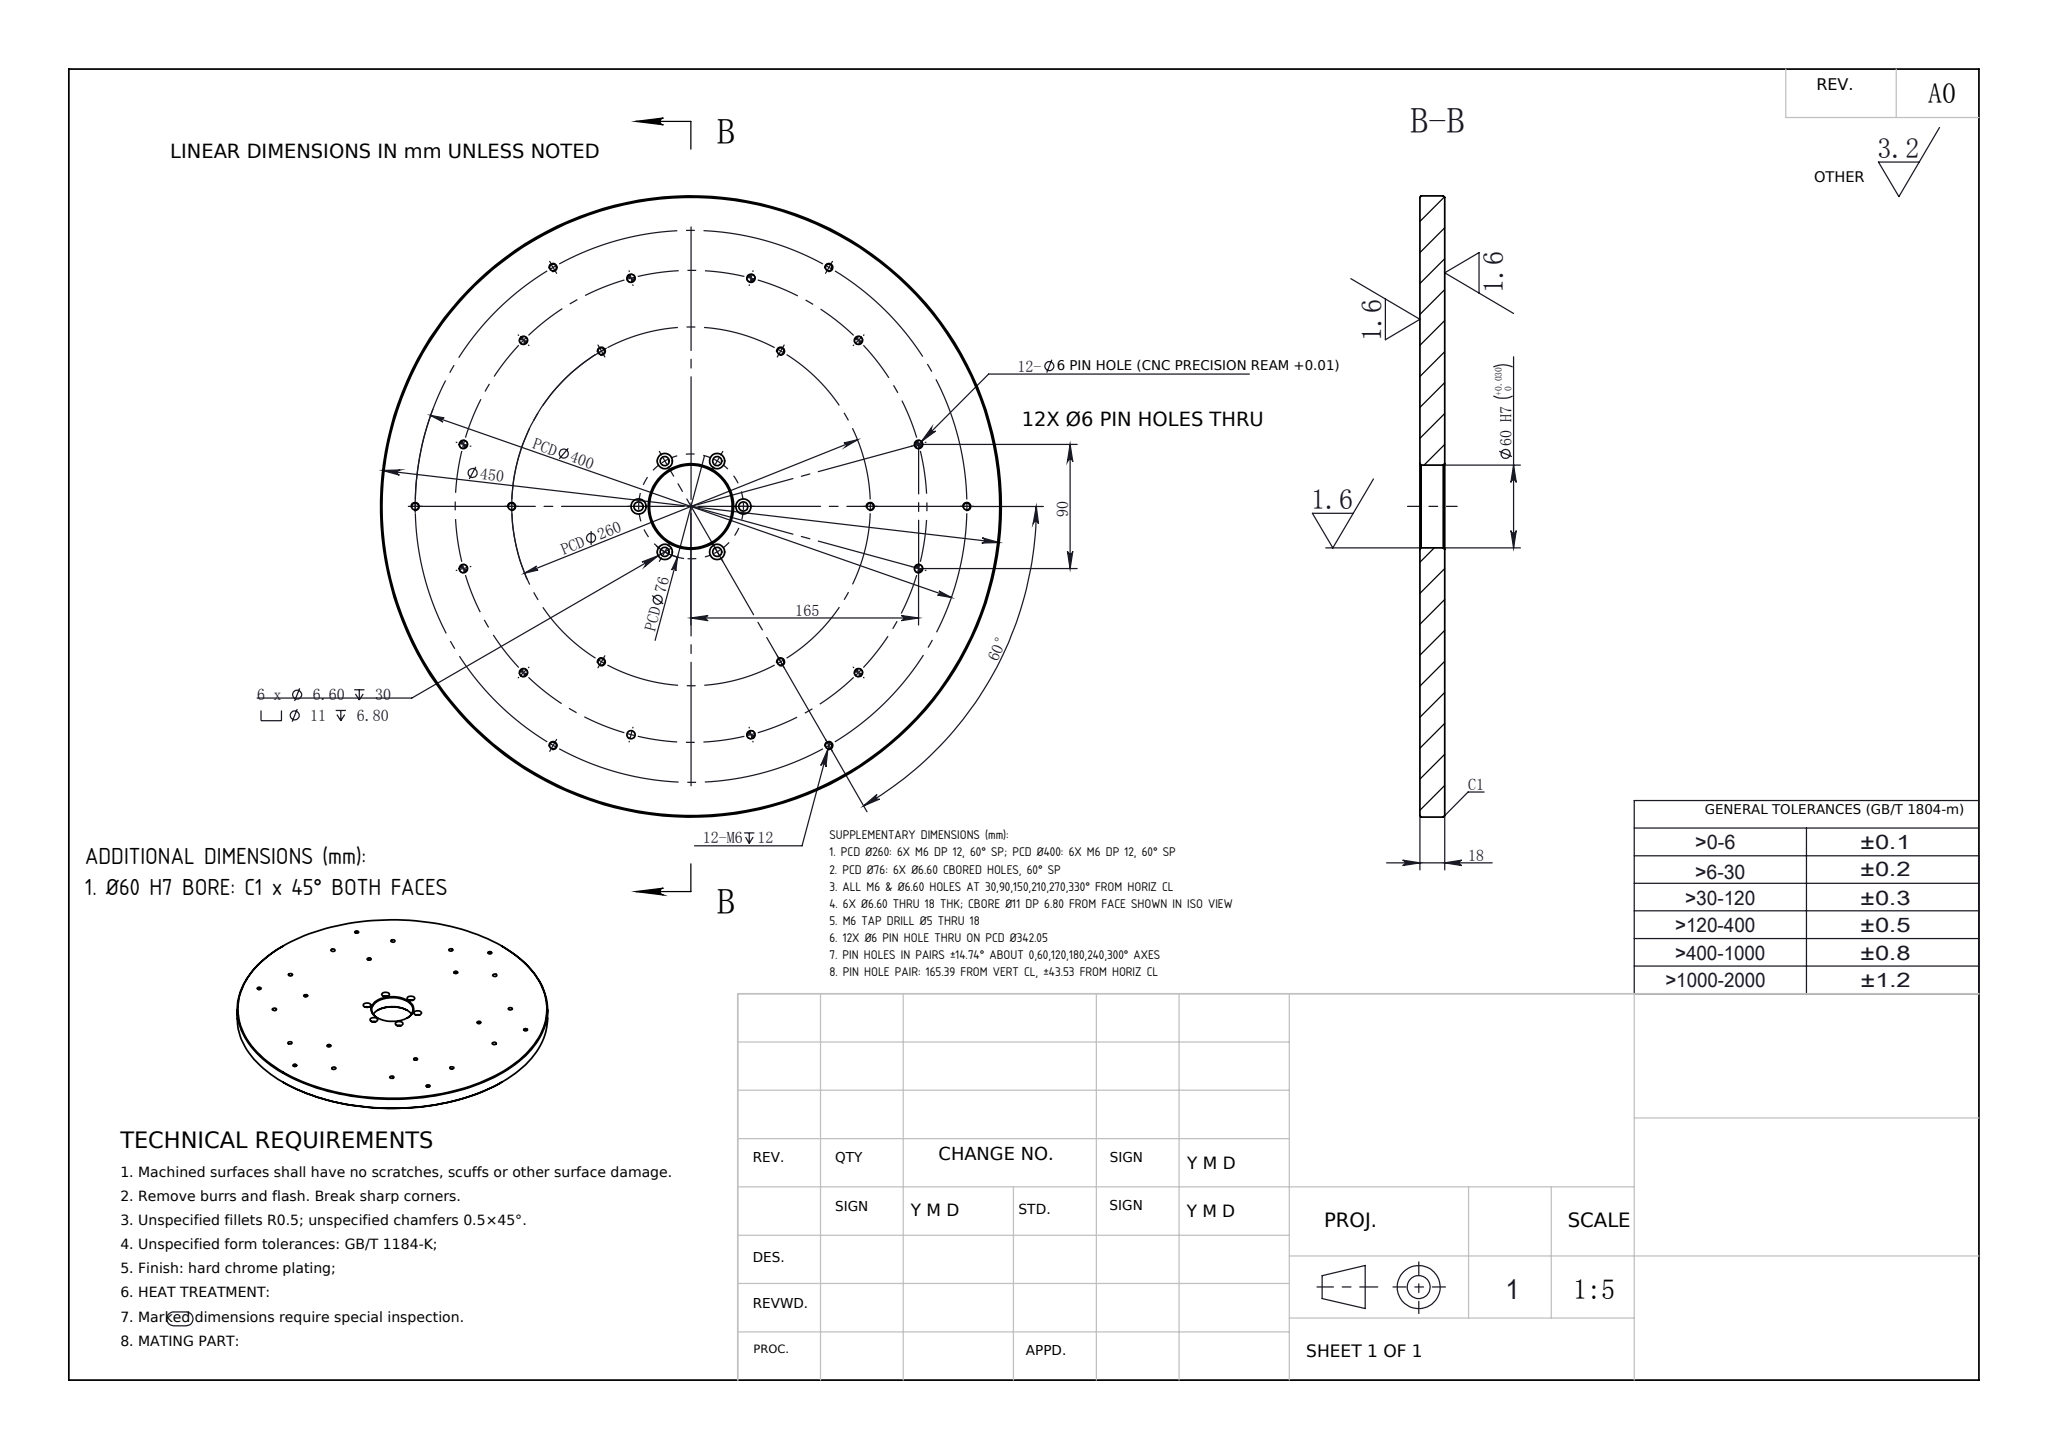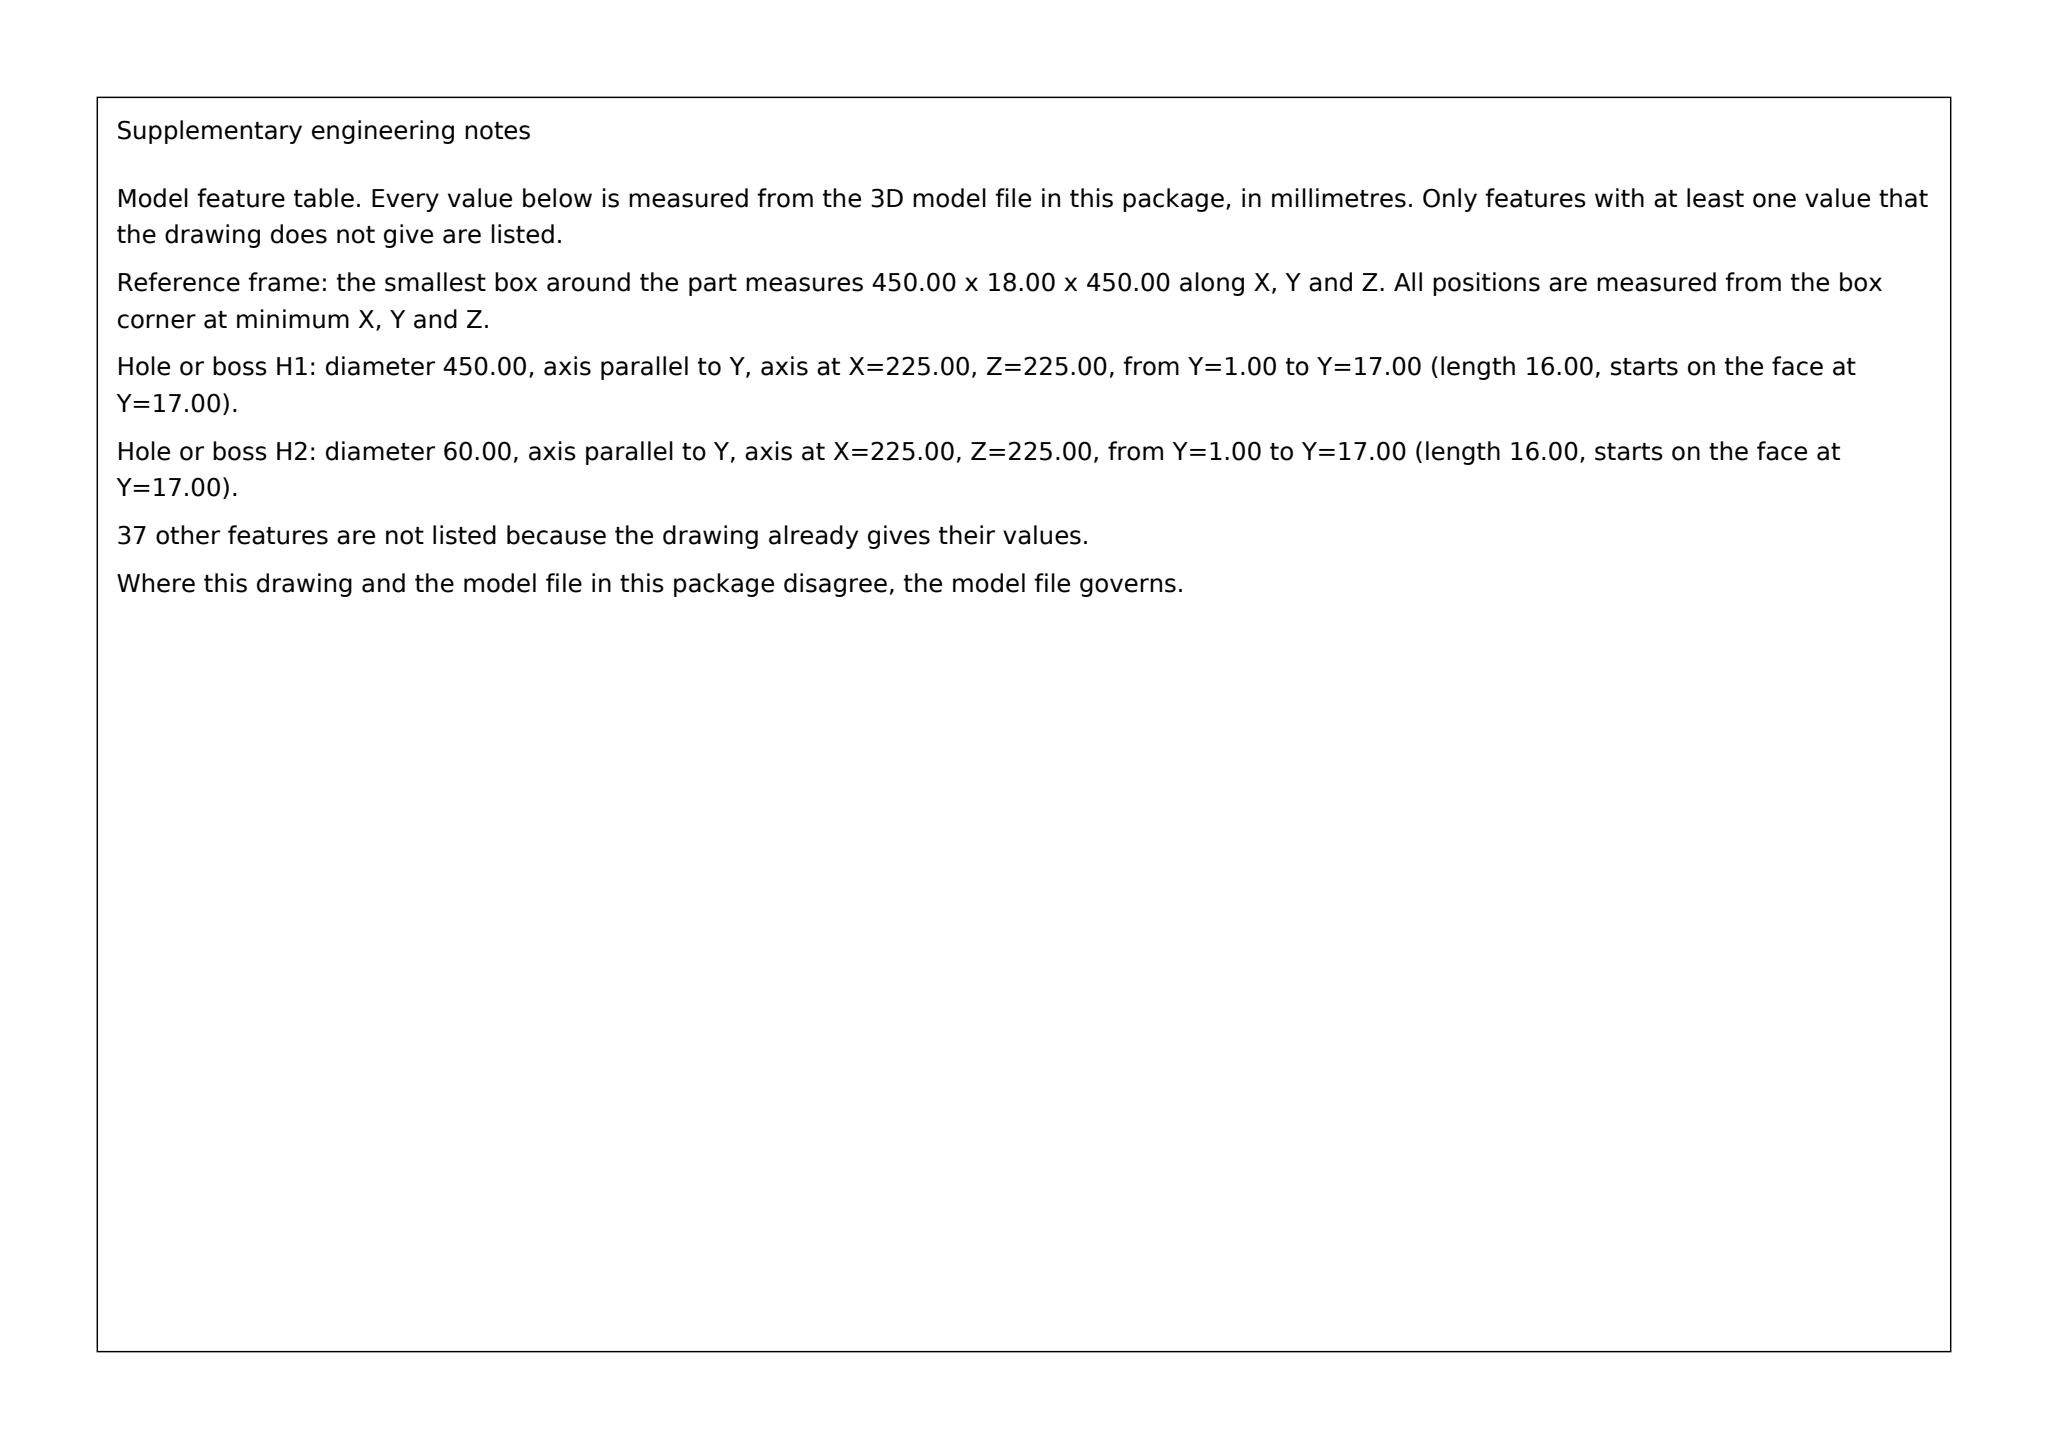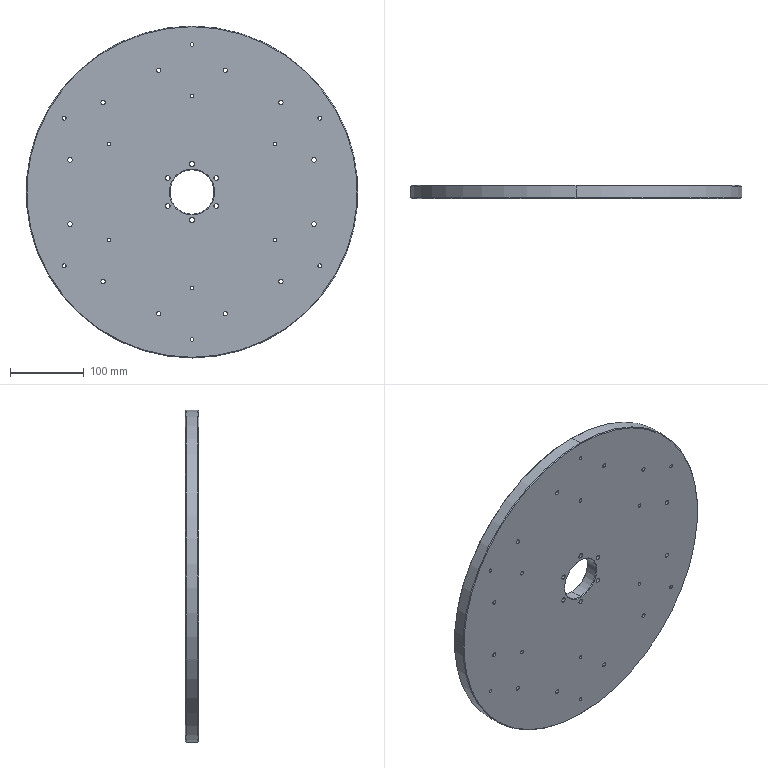Part | SolidWorks | mm | 1 solid | 92 faces | box 450 x 18 x 450 mm | volume 2793755 mm3 | cylinder 76 | cone 8 | plane 8 | commonest cylinder face diameters 5 x24 6 x24 11 x12 6.6 x12 60 x2 450 x2
build123d program:
from build123d import *

# Parameters (mm, degrees)
SKETCH1_R                  = 225
EXTRUDE1_DEPTH             = 18
SKETCH2_R                  = 3
CUT_EXTRUDE1_DEPTH         = 319.707
CIRPATTERN1_COUNT          = 6
SKETCH3_R                  = 30
EXTRUDE2_DEPTH             = 319.707
M6_TAPPED_HOLE1_AT_2_COUNT = 2
M6_TAPPED_HOLE1_AT_2_PITCH = 70
CIRPATTERN2_COUNT          = 6
CHAMFER1_SIZE              = 1
CIRPATTERN3_COUNT          = 6


with BuildPart() as part:
    # Sketch1 → Extrude1 (new body)
    with BuildSketch(Plane(origin=(0, 0, 0), x_dir=(1, 0, 0), z_dir=(0, 1, 0))):
        with Locations(Location((0, 0, 0), (0, 0, 270))):
            Circle(SKETCH1_R)
    extrude(amount=EXTRUDE1_DEPTH)

    # Sketch2 → Cut-Extrude1 (cut, through all)
    with BuildSketch(Plane(origin=(0, 18, 0), x_dir=(1, 0, 0), z_dir=(0, 1, 0))):
        with Locations(Location((-45, -165, 0), (0, 0, 270))):
            Circle(SKETCH2_R)
        with Locations(Location((45, -165, 0), (0, 0, 270))):
            Circle(SKETCH2_R)
    cut_extrude1 = extrude(amount=-CUT_EXTRUDE1_DEPTH, mode=Mode.SUBTRACT)

    # CirPattern1: Cut-Extrude1 ×6 about axis
    cirpattern1_axis = Axis((0, 0, 0), (0, 1, 0))
    for i in range(1, CIRPATTERN1_COUNT):
        add(cut_extrude1.rotate(cirpattern1_axis, i * 360 / CIRPATTERN1_COUNT), mode=Mode.SUBTRACT)

    # Sketch3 → Extrude2 (cut, through all)
    with BuildSketch(Plane(origin=(0, 18, 0), x_dir=(1, 0, 0), z_dir=(0, 1, 0))):
        with Locations(Location((0, 0, 0), (0, 0, 270))):
            Circle(SKETCH3_R)
    extrude(amount=-EXTRUDE2_DEPTH, mode=Mode.SUBTRACT)

    # Sketch4 → M6 Tapped Hole1 (revolve, cut)
    with BuildSketch(Plane(origin=(0, 18, -130), x_dir=(0, 0, 1), z_dir=(1, 0, 0))):
        Polygon((0, 0), (0, 19.502), (2.5, 18), (2.5, 0), align=None)
    m6_tapped_hole1 = revolve(axis=Axis((0, 24.35, -130), (0, -1, 0)), mode=Mode.SUBTRACT)

    # M6 Tapped Hole1 at 2: M6 Tapped Hole1 ×2
    with Locations(*[(0, 0, -i * M6_TAPPED_HOLE1_AT_2_PITCH) for i in range(1, M6_TAPPED_HOLE1_AT_2_COUNT)]):
        add(m6_tapped_hole1, mode=Mode.SUBTRACT)

    # CirPattern2: M6 Tapped Hole1 ×6 about axis
    cirpattern2_axis = Axis((0, 0, 0), (0, 1, 0))
    for i in range(1, CIRPATTERN2_COUNT):
        add(m6_tapped_hole1.rotate(cirpattern2_axis, i * 360 / CIRPATTERN2_COUNT), mode=Mode.SUBTRACT)

    # CirPattern2 copy 1 sketch → CirPattern2 copy 1 (revolve, cut)
    with BuildSketch(Plane(origin=(-173.205, 18, -100), x_dir=(0.866, 0, 0.5), z_dir=(0.5, 0, -0.866))):
        Polygon((0, 0), (0, 19.502), (2.5, 18), (2.5, 0), align=None)
    revolve(axis=Axis((-173.205, 24.35, -100), (0, -1, 0)), mode=Mode.SUBTRACT)

    # CirPattern2 copy 2 sketch → CirPattern2 copy 2 (revolve, cut)
    with BuildSketch(Plane(origin=(-173.205, 18, 100), x_dir=(0.866, 0, -0.5), z_dir=(-0.5, 0, -0.866))):
        Polygon((0, 0), (0, 19.502), (2.5, 18), (2.5, 0), align=None)
    revolve(axis=Axis((-173.205, 24.35, 100), (0, -1, 0)), mode=Mode.SUBTRACT)

    # CirPattern2 copy 3 sketch → CirPattern2 copy 3 (revolve, cut)
    with BuildSketch(Plane(origin=(0, 18, 200), x_dir=(0, 0, -1), z_dir=(-1, 0, 0))):
        Polygon((0, 0), (0, 19.502), (2.5, 18), (2.5, 0), align=None)
    revolve(axis=Axis((0, 24.35, 200), (0, -1, 0)), mode=Mode.SUBTRACT)

    # CirPattern2 copy 4 sketch → CirPattern2 copy 4 (revolve, cut)
    with BuildSketch(Plane(origin=(173.205, 18, 100), x_dir=(-0.866, 0, -0.5), z_dir=(-0.5, 0, 0.866))):
        Polygon((0, 0), (0, 19.502), (2.5, 18), (2.5, 0), align=None)
    revolve(axis=Axis((173.205, 24.35, 100), (0, -1, 0)), mode=Mode.SUBTRACT)

    # CirPattern2 copy 5 sketch → CirPattern2 copy 5 (revolve, cut)
    with BuildSketch(Plane(origin=(173.205, 18, -100), x_dir=(-0.866, 0, 0.5), z_dir=(0.5, 0, 0.866))):
        Polygon((0, 0), (0, 19.502), (2.5, 18), (2.5, 0), align=None)
    revolve(axis=Axis((173.205, 24.35, -100), (0, -1, 0)), mode=Mode.SUBTRACT)

    # Chamfer1
    chamfer1_edges = [part.edges().sort_by_distance(p)[0] for p in [
        (0, 0, -225),
        (0, 18, -225),
        (0, 0, -30),
        (0, 18, -30),
    ]]
    chamfer(chamfer1_edges, length=CHAMFER1_SIZE)

    # Sketch6 → Hole Size _ according to_ Type of Hexago (revolve, cut)
    with BuildSketch(Plane(origin=(0, 18, -38), x_dir=(0, 0, 1), z_dir=(1, 0, 0))):
        Polygon((0, 0), (0, 31.983), (3.3, 30), (3.3, 6.8), (5.5, 6.8), (5.5, 0), align=None)
    hole_size_according_to_type_of_hexago = revolve(axis=Axis((0, 24.35, -38), (0, -1, 0)), mode=Mode.SUBTRACT)

    # CirPattern3: Hole Size _ according to_ Type of Hexago ×6 about axis
    cirpattern3_axis = Axis((0, 0, 0), (0, 1, 0))
    for i in range(1, CIRPATTERN3_COUNT):
        add(hole_size_according_to_type_of_hexago.rotate(cirpattern3_axis, i * 360 / CIRPATTERN3_COUNT), mode=Mode.SUBTRACT)


solid = part.part